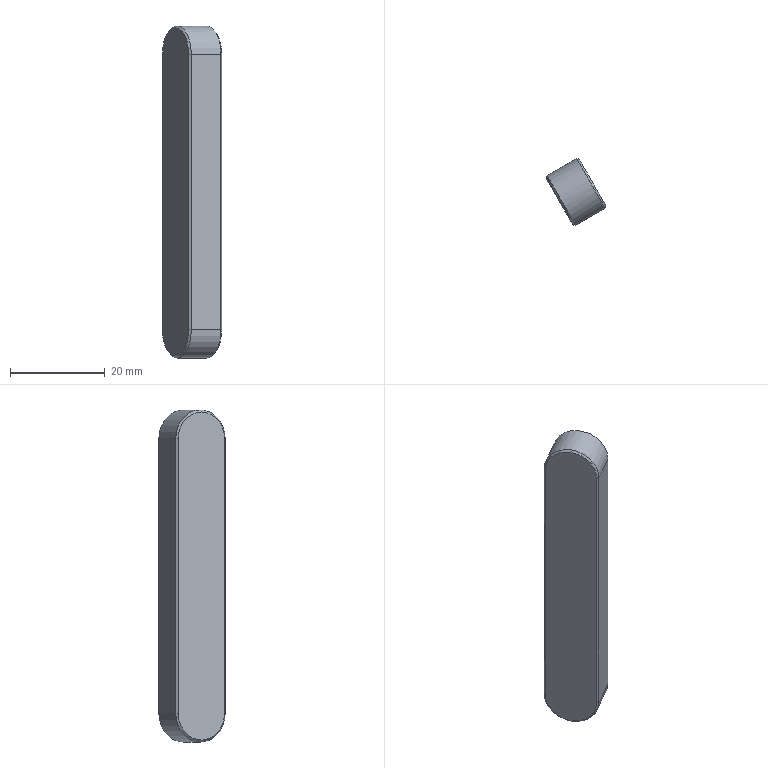Component | SolidWorks | Key12-8-70-1 | 1 solid | 17 faces | box 12.5 x 13.99 x 70 mm | volume 6448 mm3 | plane 8 | cone 6 | cylinder 3 | commonest cylinder face diameters 12 x3
build123d program:
from build123d import *

# Parameters (mm, degrees)
BOSS_EXTRUDE1_DEPTH = 8
CHAMFER1_SIZE2      = 0.4
CHAMFER1_SIZE       = 0.4


with BuildPart() as part:
    # Sketch1 → Boss-Extrude1 (new body)
    with BuildSketch(Plane(origin=(0, 0, 4), x_dir=(1, 0, 0), z_dir=(0, -1, 0))):
        with BuildLine():
            Line((-6, 54), (-6, -4))
            ThreePointArc((-6, -4), (0, -10), (6, -4))
            Line((6, -4), (6, 54))
            ThreePointArc((6, 54), (0, 60), (-6, 54))
        make_face()
    extrude(amount=-BOSS_EXTRUDE1_DEPTH)

    # Chamfer1
    chamfer1_edges = [part.edges().sort_by_distance(p)[0] for p in [
        (0, 8, -6),
        (6, 8, 29),
        (0, 8, 64),
        (6, 0, 29),
        (0, 0, -6),
        (-6, 0, 29),
        (0, 0, 64),
        (-6, 8, 29),
    ]]
    chamfer(chamfer1_edges, length=CHAMFER1_SIZE, length2=CHAMFER1_SIZE2)


solid = part.part

# Placed as in the assembly
solid = solid.moved(Location((-50.674, -11.79, -169.75), (-180, 0, -119.696)))
STEP:
#1=CARTESIAN_POINT('',(-1.721,-0.3082,-9.187));
#2=VERTEX_POINT('',#1);
#3=CARTESIAN_POINT('',(-1.831,-0.1166,-8.967));
#4=VERTEX_POINT('',#3);
#5=CARTESIAN_POINT('',(-1.721,-0.3082,-8.967));
#6=DIRECTION('',(0.8687,0.4954,0.));
#7=DIRECTION('',(0.,-0.,-1.));
#8=AXIS2_PLACEMENT_3D('',#5,#6,#7);
#9=CIRCLE('',#8,0.2205);
#10=EDGE_CURVE('',#2,#4,#9,.T.);
#11=ORIENTED_EDGE('',*,*,#10,.F.);
#12=CARTESIAN_POINT('',(-1.735,-0.316,-9.203));
#13=VERTEX_POINT('',#12);
#14=CARTESIAN_POINT('',(-1.735,-0.316,-9.203));
#15=DIRECTION('',(-0.6142,-0.3503,-0.7071));
#16=VECTOR('',#15,39.37);
#17=LINE('',#14,#16);
#18=EDGE_CURVE('',#2,#13,#17,.T.);
#19=ORIENTED_EDGE('',*,*,#18,.T.);
#20=CARTESIAN_POINT('',(-1.852,-0.1108,-8.967));
#21=VERTEX_POINT('',#20);
#22=CARTESIAN_POINT('',(-1.735,-0.316,-8.967));
#23=DIRECTION('',(-0.8687,-0.4954,-0.));
#24=DIRECTION('',(0.,0.,-1.));
#25=AXIS2_PLACEMENT_3D('',#22,#23,#24);
#26=CIRCLE('',#25,0.2362);
#27=EDGE_CURVE('',#21,#13,#26,.T.);
#28=ORIENTED_EDGE('',*,*,#27,.F.);
#29=CARTESIAN_POINT('',(-1.831,-0.1166,-8.967));
#30=DIRECTION('',(-0.9645,0.2639,-0.));
#31=VECTOR('',#30,39.37);
#32=LINE('',#29,#31);
#33=EDGE_CURVE('',#4,#21,#32,.T.);
#34=ORIENTED_EDGE('',*,*,#33,.F.);
#35=EDGE_LOOP('',(#11,#19,#28,#34));
#36=FACE_OUTER_BOUND('',#35,.T.);
#37=CARTESIAN_POINT('',(-1.735,-0.316,-8.967));
#38=DIRECTION('',(-0.8687,-0.4954,-0.));
#39=DIRECTION('',(0.,0.,-1.));
#40=AXIS2_PLACEMENT_3D('',#37,#38,#39);
#41=CONICAL_SURFACE('',#40,0.2362,0.7854);
#42=ADVANCED_FACE('',(#36),#41,.T.);
#43=CARTESIAN_POINT('',(-1.995,-0.4642,-6.463));
#44=VERTEX_POINT('',#43);
#45=CARTESIAN_POINT('',(-2.104,-0.2727,-6.683));
#46=VERTEX_POINT('',#45);
#47=CARTESIAN_POINT('',(-1.995,-0.4642,-6.683));
#48=DIRECTION('',(-0.8687,-0.4954,-0.));
#49=DIRECTION('',(0.,0.,-1.));
#50=AXIS2_PLACEMENT_3D('',#47,#48,#49);
#51=CIRCLE('',#50,0.2205);
#52=EDGE_CURVE('',#44,#46,#51,.T.);
#53=ORIENTED_EDGE('',*,*,#52,.F.);
#54=CARTESIAN_POINT('',(-1.981,-0.4564,-6.447));
#55=VERTEX_POINT('',#54);
#56=CARTESIAN_POINT('',(-1.995,-0.4642,-6.463));
#57=DIRECTION('',(0.6142,0.3503,0.7071));
#58=VECTOR('',#57,39.37);
#59=LINE('',#56,#58);
#60=EDGE_CURVE('',#44,#55,#59,.T.);
#61=ORIENTED_EDGE('',*,*,#60,.T.);
#62=CARTESIAN_POINT('',(-2.098,-0.2512,-6.683));
#63=VERTEX_POINT('',#62);
#64=CARTESIAN_POINT('',(-1.981,-0.4564,-6.683));
#65=DIRECTION('',(0.8687,0.4954,0.));
#66=DIRECTION('',(0.,0.,-1.));
#67=AXIS2_PLACEMENT_3D('',#64,#65,#66);
#68=CIRCLE('',#67,0.2362);
#69=EDGE_CURVE('',#63,#55,#68,.T.);
#70=ORIENTED_EDGE('',*,*,#69,.F.);
#71=CARTESIAN_POINT('',(-2.098,-0.2512,-6.683));
#72=DIRECTION('',(-0.2639,-0.9645,-0.));
#73=VECTOR('',#72,39.37);
#74=LINE('',#71,#73);
#75=EDGE_CURVE('',#63,#46,#74,.T.);
#76=ORIENTED_EDGE('',*,*,#75,.T.);
#77=EDGE_LOOP('',(#53,#61,#70,#76));
#78=FACE_OUTER_BOUND('',#77,.T.);
#79=CARTESIAN_POINT('',(-1.995,-0.4642,-6.683));
#80=DIRECTION('',(0.8687,0.4954,0.));
#81=DIRECTION('',(-0.,0.,1.));
#82=AXIS2_PLACEMENT_3D('',#79,#80,#81);
#83=CONICAL_SURFACE('',#82,0.2205,0.7854);
#84=ADVANCED_FACE('',(#78),#83,.T.);
#85=ORIENTED_EDGE('',*,*,#27,.T.);
#86=CARTESIAN_POINT('',(-1.981,-0.4564,-9.203));
#87=VERTEX_POINT('',#86);
#88=CARTESIAN_POINT('',(-1.721,-0.3082,-9.203));
#89=DIRECTION('',(-0.8687,-0.4954,-0.));
#90=VECTOR('',#89,39.37);
#91=LINE('',#88,#90);
#92=EDGE_CURVE('',#13,#87,#91,.T.);
#93=ORIENTED_EDGE('',*,*,#92,.T.);
#94=CARTESIAN_POINT('',(-2.098,-0.2512,-8.967));
#95=VERTEX_POINT('',#94);
#96=CARTESIAN_POINT('',(-1.981,-0.4564,-8.967));
#97=DIRECTION('',(0.8687,0.4954,0.));
#98=DIRECTION('',(0.,0.,-1.));
#99=AXIS2_PLACEMENT_3D('',#96,#97,#98);
#100=CIRCLE('',#99,0.2362);
#101=EDGE_CURVE('',#87,#95,#100,.T.);
#102=ORIENTED_EDGE('',*,*,#101,.T.);
#103=CARTESIAN_POINT('',(-1.838,-0.103,-8.967));
#104=DIRECTION('',(-0.8687,-0.4954,-0.));
#105=VECTOR('',#104,39.37);
#106=LINE('',#103,#105);
#107=EDGE_CURVE('',#21,#95,#106,.T.);
#108=ORIENTED_EDGE('',*,*,#107,.F.);
#109=EDGE_LOOP('',(#85,#93,#102,#108));
#110=FACE_OUTER_BOUND('',#109,.T.);
#111=CARTESIAN_POINT('',(-1.721,-0.3082,-8.967));
#112=DIRECTION('',(-0.8687,-0.4954,-0.));
#113=DIRECTION('',(0.,0.,-1.));
#114=AXIS2_PLACEMENT_3D('',#111,#112,#113);
#115=CYLINDRICAL_SURFACE('',#114,0.2362);
#116=ADVANCED_FACE('',(#110),#115,.T.);
#117=CARTESIAN_POINT('',(-1.852,-0.1108,-6.683));
#118=VERTEX_POINT('',#117);
#119=CARTESIAN_POINT('',(-1.838,-0.103,-6.683));
#120=DIRECTION('',(-0.8687,-0.4954,-0.));
#121=VECTOR('',#120,39.37);
#122=LINE('',#119,#121);
#123=EDGE_CURVE('',#118,#63,#122,.T.);
#124=ORIENTED_EDGE('',*,*,#123,.T.);
#125=ORIENTED_EDGE('',*,*,#69,.T.);
#126=CARTESIAN_POINT('',(-1.864,-0.6616,-6.683));
#127=VERTEX_POINT('',#126);
#128=CARTESIAN_POINT('',(-1.981,-0.4564,-6.683));
#129=DIRECTION('',(0.8687,0.4954,0.));
#130=DIRECTION('',(0.,-0.,-1.));
#131=AXIS2_PLACEMENT_3D('',#128,#129,#130);
#132=CIRCLE('',#131,0.2362);
#133=EDGE_CURVE('',#55,#127,#132,.T.);
#134=ORIENTED_EDGE('',*,*,#133,.T.);
#135=CARTESIAN_POINT('',(-1.618,-0.5212,-6.683));
#136=VERTEX_POINT('',#135);
#137=CARTESIAN_POINT('',(-1.604,-0.5134,-6.683));
#138=DIRECTION('',(-0.8687,-0.4954,-0.));
#139=VECTOR('',#138,39.37);
#140=LINE('',#137,#139);
#141=EDGE_CURVE('',#136,#127,#140,.T.);
#142=ORIENTED_EDGE('',*,*,#141,.F.);
#143=CARTESIAN_POINT('',(-1.735,-0.316,-6.683));
#144=DIRECTION('',(-0.8687,-0.4954,-0.));
#145=DIRECTION('',(0.,0.,-1.));
#146=AXIS2_PLACEMENT_3D('',#143,#144,#145);
#147=CIRCLE('',#146,0.2362);
#148=EDGE_CURVE('',#136,#118,#147,.T.);
#149=ORIENTED_EDGE('',*,*,#148,.T.);
#150=EDGE_LOOP('',(#124,#125,#134,#142,#149));
#151=FACE_OUTER_BOUND('',#150,.T.);
#152=CARTESIAN_POINT('',(-1.721,-0.3082,-6.683));
#153=DIRECTION('',(-0.8687,-0.4954,-0.));
#154=DIRECTION('',(0.,0.,-1.));
#155=AXIS2_PLACEMENT_3D('',#152,#153,#154);
#156=CYLINDRICAL_SURFACE('',#155,0.2362);
#157=ADVANCED_FACE('',(#151),#156,.T.);
#158=ORIENTED_EDGE('',*,*,#141,.T.);
#159=CARTESIAN_POINT('',(-1.864,-0.6616,-8.967));
#160=VERTEX_POINT('',#159);
#161=CARTESIAN_POINT('',(-1.864,-0.6616,-8.967));
#162=DIRECTION('',(0.,0.,-1.));
#163=VECTOR('',#162,39.37);
#164=LINE('',#161,#163);
#165=EDGE_CURVE('',#127,#160,#164,.T.);
#166=ORIENTED_EDGE('',*,*,#165,.T.);
#167=CARTESIAN_POINT('',(-1.618,-0.5212,-8.967));
#168=VERTEX_POINT('',#167);
#169=CARTESIAN_POINT('',(-1.604,-0.5134,-8.967));
#170=DIRECTION('',(-0.8687,-0.4954,-0.));
#171=VECTOR('',#170,39.37);
#172=LINE('',#169,#171);
#173=EDGE_CURVE('',#168,#160,#172,.T.);
#174=ORIENTED_EDGE('',*,*,#173,.F.);
#175=CARTESIAN_POINT('',(-1.618,-0.5212,-6.683));
#176=DIRECTION('',(-0.,-0.,1.));
#177=VECTOR('',#176,39.37);
#178=LINE('',#175,#177);
#179=EDGE_CURVE('',#168,#136,#178,.T.);
#180=ORIENTED_EDGE('',*,*,#179,.T.);
#181=EDGE_LOOP('',(#158,#166,#174,#180));
#182=FACE_OUTER_BOUND('',#181,.T.);
#183=CARTESIAN_POINT('',(-1.604,-0.5134,-8.967));
#184=DIRECTION('',(0.4954,-0.8687,0.));
#185=DIRECTION('',(0.,0.,-1.));
#186=AXIS2_PLACEMENT_3D('',#183,#184,#185);
#187=PLANE('',#186);
#188=ADVANCED_FACE('',(#182),#187,.T.);
#189=ORIENTED_EDGE('',*,*,#92,.F.);
#190=CARTESIAN_POINT('',(-1.735,-0.316,-8.967));
#191=DIRECTION('',(-0.8687,-0.4954,-0.));
#192=DIRECTION('',(0.,0.,-1.));
#193=AXIS2_PLACEMENT_3D('',#190,#191,#192);
#194=CIRCLE('',#193,0.2362);
#195=EDGE_CURVE('',#13,#168,#194,.T.);
#196=ORIENTED_EDGE('',*,*,#195,.T.);
#197=ORIENTED_EDGE('',*,*,#173,.T.);
#198=CARTESIAN_POINT('',(-1.981,-0.4564,-8.967));
#199=DIRECTION('',(0.8687,0.4954,0.));
#200=DIRECTION('',(0.,0.,-1.));
#201=AXIS2_PLACEMENT_3D('',#198,#199,#200);
#202=CIRCLE('',#201,0.2362);
#203=EDGE_CURVE('',#160,#87,#202,.T.);
#204=ORIENTED_EDGE('',*,*,#203,.T.);
#205=EDGE_LOOP('',(#189,#196,#197,#204));
#206=FACE_OUTER_BOUND('',#205,.T.);
#207=CARTESIAN_POINT('',(-1.721,-0.3082,-8.967));
#208=DIRECTION('',(-0.8687,-0.4954,-0.));
#209=DIRECTION('',(0.,0.,-1.));
#210=AXIS2_PLACEMENT_3D('',#207,#208,#209);
#211=CYLINDRICAL_SURFACE('',#210,0.2362);
#212=ADVANCED_FACE('',(#206),#211,.T.);
#213=ORIENTED_EDGE('',*,*,#107,.T.);
#214=CARTESIAN_POINT('',(-2.098,-0.2512,-6.683));
#215=DIRECTION('',(-0.,-0.,1.));
#216=VECTOR('',#215,39.37);
#217=LINE('',#214,#216);
#218=EDGE_CURVE('',#95,#63,#217,.T.);
#219=ORIENTED_EDGE('',*,*,#218,.T.);
#220=ORIENTED_EDGE('',*,*,#123,.F.);
#221=CARTESIAN_POINT('',(-1.852,-0.1108,-8.967));
#222=DIRECTION('',(0.,0.,-1.));
#223=VECTOR('',#222,39.37);
#224=LINE('',#221,#223);
#225=EDGE_CURVE('',#118,#21,#224,.T.);
#226=ORIENTED_EDGE('',*,*,#225,.T.);
#227=EDGE_LOOP('',(#213,#219,#220,#226));
#228=FACE_OUTER_BOUND('',#227,.T.);
#229=CARTESIAN_POINT('',(-1.838,-0.103,-6.683));
#230=DIRECTION('',(-0.4954,0.8687,-0.));
#231=DIRECTION('',(-0.,-0.,1.));
#232=AXIS2_PLACEMENT_3D('',#229,#230,#231);
#233=PLANE('',#232);
#234=ADVANCED_FACE('',(#228),#233,.T.);
#235=CARTESIAN_POINT('',(-1.612,-0.4997,-8.967));
#236=VERTEX_POINT('',#235);
#237=CARTESIAN_POINT('',(-1.721,-0.3082,-8.967));
#238=DIRECTION('',(0.8687,0.4954,0.));
#239=DIRECTION('',(0.,0.,-1.));
#240=AXIS2_PLACEMENT_3D('',#237,#238,#239);
#241=CIRCLE('',#240,0.2205);
#242=EDGE_CURVE('',#236,#2,#241,.T.);
#243=ORIENTED_EDGE('',*,*,#242,.T.);
#244=ORIENTED_EDGE('',*,*,#10,.T.);
#245=CARTESIAN_POINT('',(-1.831,-0.1166,-6.683));
#246=VERTEX_POINT('',#245);
#247=CARTESIAN_POINT('',(-1.831,-0.1166,-6.683));
#248=DIRECTION('',(-0.,-0.,1.));
#249=VECTOR('',#248,39.37);
#250=LINE('',#247,#249);
#251=EDGE_CURVE('',#4,#246,#250,.T.);
#252=ORIENTED_EDGE('',*,*,#251,.T.);
#253=CARTESIAN_POINT('',(-1.612,-0.4997,-6.683));
#254=VERTEX_POINT('',#253);
#255=CARTESIAN_POINT('',(-1.721,-0.3082,-6.683));
#256=DIRECTION('',(0.8687,0.4954,0.));
#257=DIRECTION('',(0.,0.,-1.));
#258=AXIS2_PLACEMENT_3D('',#255,#256,#257);
#259=CIRCLE('',#258,0.2205);
#260=EDGE_CURVE('',#246,#254,#259,.T.);
#261=ORIENTED_EDGE('',*,*,#260,.T.);
#262=CARTESIAN_POINT('',(-1.612,-0.4997,-8.967));
#263=DIRECTION('',(0.,0.,-1.));
#264=VECTOR('',#263,39.37);
#265=LINE('',#262,#264);
#266=EDGE_CURVE('',#254,#236,#265,.T.);
#267=ORIENTED_EDGE('',*,*,#266,.T.);
#268=EDGE_LOOP('',(#243,#244,#252,#261,#267));
#269=FACE_OUTER_BOUND('',#268,.T.);
#270=CARTESIAN_POINT('',(-1.721,-0.3082,-6.683));
#271=DIRECTION('',(-0.8687,-0.4954,-0.));
#272=DIRECTION('',(0.,0.,-1.));
#273=AXIS2_PLACEMENT_3D('',#270,#271,#272);
#274=PLANE('',#273);
#275=ADVANCED_FACE('',(#269),#274,.F.);
#276=CARTESIAN_POINT('',(-2.104,-0.2727,-8.967));
#277=VERTEX_POINT('',#276);
#278=CARTESIAN_POINT('',(-1.886,-0.6557,-8.967));
#279=VERTEX_POINT('',#278);
#280=CARTESIAN_POINT('',(-1.995,-0.4642,-8.967));
#281=DIRECTION('',(-0.8687,-0.4954,-0.));
#282=DIRECTION('',(0.,0.,-1.));
#283=AXIS2_PLACEMENT_3D('',#280,#281,#282);
#284=CIRCLE('',#283,0.2205);
#285=EDGE_CURVE('',#277,#279,#284,.T.);
#286=ORIENTED_EDGE('',*,*,#285,.T.);
#287=CARTESIAN_POINT('',(-1.886,-0.6557,-6.683));
#288=VERTEX_POINT('',#287);
#289=CARTESIAN_POINT('',(-1.886,-0.6557,-6.683));
#290=DIRECTION('',(-0.,-0.,1.));
#291=VECTOR('',#290,39.37);
#292=LINE('',#289,#291);
#293=EDGE_CURVE('',#279,#288,#292,.T.);
#294=ORIENTED_EDGE('',*,*,#293,.T.);
#295=CARTESIAN_POINT('',(-1.995,-0.4642,-6.683));
#296=DIRECTION('',(-0.8687,-0.4954,-0.));
#297=DIRECTION('',(0.,0.,-1.));
#298=AXIS2_PLACEMENT_3D('',#295,#296,#297);
#299=CIRCLE('',#298,0.2205);
#300=EDGE_CURVE('',#288,#44,#299,.T.);
#301=ORIENTED_EDGE('',*,*,#300,.T.);
#302=ORIENTED_EDGE('',*,*,#52,.T.);
#303=CARTESIAN_POINT('',(-2.104,-0.2727,-6.683));
#304=DIRECTION('',(0.,0.,-1.));
#305=VECTOR('',#304,39.37);
#306=LINE('',#303,#305);
#307=EDGE_CURVE('',#46,#277,#306,.T.);
#308=ORIENTED_EDGE('',*,*,#307,.T.);
#309=EDGE_LOOP('',(#286,#294,#301,#302,#308));
#310=FACE_OUTER_BOUND('',#309,.T.);
#311=CARTESIAN_POINT('',(-1.995,-0.4642,-6.683));
#312=DIRECTION('',(-0.8687,-0.4954,-0.));
#313=DIRECTION('',(0.,0.,-1.));
#314=AXIS2_PLACEMENT_3D('',#311,#312,#313);
#315=PLANE('',#314);
#316=ADVANCED_FACE('',(#310),#315,.T.);
#317=ORIENTED_EDGE('',*,*,#75,.F.);
#318=ORIENTED_EDGE('',*,*,#218,.F.);
#319=CARTESIAN_POINT('',(-2.104,-0.2727,-8.967));
#320=DIRECTION('',(0.2639,0.9645,0.));
#321=VECTOR('',#320,39.37);
#322=LINE('',#319,#321);
#323=EDGE_CURVE('',#277,#95,#322,.T.);
#324=ORIENTED_EDGE('',*,*,#323,.F.);
#325=ORIENTED_EDGE('',*,*,#307,.F.);
#326=EDGE_LOOP('',(#317,#318,#324,#325));
#327=FACE_OUTER_BOUND('',#326,.T.);
#328=CARTESIAN_POINT('',(-2.104,-0.2727,-6.683));
#329=DIRECTION('',(0.9645,-0.2639,0.));
#330=DIRECTION('',(0.,0.,-1.));
#331=AXIS2_PLACEMENT_3D('',#328,#329,#330);
#332=PLANE('',#331);
#333=ADVANCED_FACE('',(#327),#332,.F.);
#334=ORIENTED_EDGE('',*,*,#323,.T.);
#335=ORIENTED_EDGE('',*,*,#101,.F.);
#336=ORIENTED_EDGE('',*,*,#203,.F.);
#337=CARTESIAN_POINT('',(-1.886,-0.6557,-8.967));
#338=DIRECTION('',(0.9645,-0.2639,0.));
#339=VECTOR('',#338,39.37);
#340=LINE('',#337,#339);
#341=EDGE_CURVE('',#279,#160,#340,.T.);
#342=ORIENTED_EDGE('',*,*,#341,.F.);
#343=ORIENTED_EDGE('',*,*,#285,.F.);
#344=EDGE_LOOP('',(#334,#335,#336,#342,#343));
#345=FACE_OUTER_BOUND('',#344,.T.);
#346=CARTESIAN_POINT('',(-1.995,-0.4642,-8.967));
#347=DIRECTION('',(0.8687,0.4954,0.));
#348=DIRECTION('',(-0.,0.,1.));
#349=AXIS2_PLACEMENT_3D('',#346,#347,#348);
#350=CONICAL_SURFACE('',#349,0.2205,0.7854);
#351=ADVANCED_FACE('',(#345),#350,.T.);
#352=ORIENTED_EDGE('',*,*,#60,.F.);
#353=ORIENTED_EDGE('',*,*,#300,.F.);
#354=CARTESIAN_POINT('',(-1.864,-0.6616,-6.683));
#355=DIRECTION('',(-0.9645,0.2639,-0.));
#356=VECTOR('',#355,39.37);
#357=LINE('',#354,#356);
#358=EDGE_CURVE('',#127,#288,#357,.T.);
#359=ORIENTED_EDGE('',*,*,#358,.F.);
#360=ORIENTED_EDGE('',*,*,#133,.F.);
#361=EDGE_LOOP('',(#352,#353,#359,#360));
#362=FACE_OUTER_BOUND('',#361,.T.);
#363=CARTESIAN_POINT('',(-1.995,-0.4642,-6.683));
#364=DIRECTION('',(0.8687,0.4954,0.));
#365=DIRECTION('',(-0.,0.,1.));
#366=AXIS2_PLACEMENT_3D('',#363,#364,#365);
#367=CONICAL_SURFACE('',#366,0.2205,0.7854);
#368=ADVANCED_FACE('',(#362),#367,.T.);
#369=ORIENTED_EDGE('',*,*,#341,.T.);
#370=ORIENTED_EDGE('',*,*,#165,.F.);
#371=ORIENTED_EDGE('',*,*,#358,.T.);
#372=ORIENTED_EDGE('',*,*,#293,.F.);
#373=EDGE_LOOP('',(#369,#370,#371,#372));
#374=FACE_OUTER_BOUND('',#373,.T.);
#375=CARTESIAN_POINT('',(-1.886,-0.6557,-6.683));
#376=DIRECTION('',(0.2639,0.9645,0.));
#377=DIRECTION('',(-0.,-0.,1.));
#378=AXIS2_PLACEMENT_3D('',#375,#376,#377);
#379=PLANE('',#378);
#380=ADVANCED_FACE('',(#374),#379,.F.);
#381=CARTESIAN_POINT('',(-1.612,-0.4997,-8.967));
#382=DIRECTION('',(-0.2639,-0.9645,-0.));
#383=VECTOR('',#382,39.37);
#384=LINE('',#381,#383);
#385=EDGE_CURVE('',#236,#168,#384,.T.);
#386=ORIENTED_EDGE('',*,*,#385,.F.);
#387=ORIENTED_EDGE('',*,*,#266,.F.);
#388=CARTESIAN_POINT('',(-1.618,-0.5212,-6.683));
#389=DIRECTION('',(0.2639,0.9645,0.));
#390=VECTOR('',#389,39.37);
#391=LINE('',#388,#390);
#392=EDGE_CURVE('',#136,#254,#391,.T.);
#393=ORIENTED_EDGE('',*,*,#392,.F.);
#394=ORIENTED_EDGE('',*,*,#179,.F.);
#395=EDGE_LOOP('',(#386,#387,#393,#394));
#396=FACE_OUTER_BOUND('',#395,.T.);
#397=CARTESIAN_POINT('',(-1.618,-0.5212,-8.967));
#398=DIRECTION('',(0.9645,-0.2639,0.));
#399=DIRECTION('',(0.,0.,-1.));
#400=AXIS2_PLACEMENT_3D('',#397,#398,#399);
#401=PLANE('',#400);
#402=ADVANCED_FACE('',(#396),#401,.T.);
#403=ORIENTED_EDGE('',*,*,#392,.T.);
#404=ORIENTED_EDGE('',*,*,#260,.F.);
#405=CARTESIAN_POINT('',(-1.852,-0.1108,-6.683));
#406=DIRECTION('',(0.9645,-0.2639,0.));
#407=VECTOR('',#406,39.37);
#408=LINE('',#405,#407);
#409=EDGE_CURVE('',#118,#246,#408,.T.);
#410=ORIENTED_EDGE('',*,*,#409,.F.);
#411=ORIENTED_EDGE('',*,*,#148,.F.);
#412=EDGE_LOOP('',(#403,#404,#410,#411));
#413=FACE_OUTER_BOUND('',#412,.T.);
#414=CARTESIAN_POINT('',(-1.735,-0.316,-6.683));
#415=DIRECTION('',(-0.8687,-0.4954,-0.));
#416=DIRECTION('',(0.,0.,-1.));
#417=AXIS2_PLACEMENT_3D('',#414,#415,#416);
#418=CONICAL_SURFACE('',#417,0.2362,0.7854);
#419=ADVANCED_FACE('',(#413),#418,.T.);
#420=ORIENTED_EDGE('',*,*,#18,.F.);
#421=ORIENTED_EDGE('',*,*,#242,.F.);
#422=ORIENTED_EDGE('',*,*,#385,.T.);
#423=ORIENTED_EDGE('',*,*,#195,.F.);
#424=EDGE_LOOP('',(#420,#421,#422,#423));
#425=FACE_OUTER_BOUND('',#424,.T.);
#426=CARTESIAN_POINT('',(-1.735,-0.316,-8.967));
#427=DIRECTION('',(-0.8687,-0.4954,-0.));
#428=DIRECTION('',(0.,0.,-1.));
#429=AXIS2_PLACEMENT_3D('',#426,#427,#428);
#430=CONICAL_SURFACE('',#429,0.2362,0.7854);
#431=ADVANCED_FACE('',(#425),#430,.T.);
#432=ORIENTED_EDGE('',*,*,#409,.T.);
#433=ORIENTED_EDGE('',*,*,#251,.F.);
#434=ORIENTED_EDGE('',*,*,#33,.T.);
#435=ORIENTED_EDGE('',*,*,#225,.F.);
#436=EDGE_LOOP('',(#432,#433,#434,#435));
#437=FACE_OUTER_BOUND('',#436,.T.);
#438=CARTESIAN_POINT('',(-1.852,-0.1108,-6.683));
#439=DIRECTION('',(0.2639,0.9645,0.));
#440=DIRECTION('',(-0.,-0.,1.));
#441=AXIS2_PLACEMENT_3D('',#438,#439,#440);
#442=PLANE('',#441);
#443=ADVANCED_FACE('',(#437),#442,.T.);
#444=CLOSED_SHELL('',(#42,#84,#116,#157,#188,#212,#234,#275,#316,#333,#351,#368,#380,#402,#419,#431,#443));
#445=MANIFOLD_SOLID_BREP('',#444);
#446=CARTESIAN_POINT('',(0.,0.,0.));
#447=DIRECTION('',(0.,0.,1.));
#448=DIRECTION('',(1.,0.,0.));
#449=AXIS2_PLACEMENT_3D('',#446,#447,#448);
#450=(LENGTH_UNIT()NAMED_UNIT(*)SI_UNIT($,.METRE.));
#451=LENGTH_MEASURE_WITH_UNIT(LENGTH_MEASURE(0.0254),#450);
#452=DIMENSIONAL_EXPONENTS(1.,0.,0.,0.,0.,0.,0.);
#453=(CONVERSION_BASED_UNIT('',#451)LENGTH_UNIT()NAMED_UNIT(#452));
#454=UNCERTAINTY_MEASURE_WITH_UNIT(LENGTH_MEASURE(0.00001),#453,'','');
#455=(NAMED_UNIT(*)PLANE_ANGLE_UNIT()SI_UNIT($,.RADIAN.));
#456=(NAMED_UNIT(*)SI_UNIT($,.STERADIAN.)SOLID_ANGLE_UNIT());
#457=(GEOMETRIC_REPRESENTATION_CONTEXT(3)GLOBAL_UNCERTAINTY_ASSIGNED_CONTEXT((#454))GLOBAL_UNIT_ASSIGNED_CONTEXT((#453,#455,#456))REPRESENTATION_CONTEXT('',''));
#458=ADVANCED_BREP_SHAPE_REPRESENTATION('',(#445,#449),#457);
#459=COLOUR_RGB('',0.7922,0.8196,0.9333);
#460=FILL_AREA_STYLE_COLOUR('',#459);
#461=FILL_AREA_STYLE('',(#460));
#462=SURFACE_STYLE_FILL_AREA(#461);
#463=SURFACE_SIDE_STYLE('',(#462));
#464=SURFACE_STYLE_USAGE(.BOTH.,#463);
#465=PRESENTATION_STYLE_ASSIGNMENT((#464));
#466=STYLED_ITEM('',(#465),#445);
#467=PRESENTATION_LAYER_ASSIGNMENT('','',(#466));
#468=(LENGTH_UNIT()NAMED_UNIT(*)SI_UNIT($,.METRE.));
#469=LENGTH_MEASURE_WITH_UNIT(LENGTH_MEASURE(0.0254),#468);
#470=DIMENSIONAL_EXPONENTS(1.,0.,0.,0.,0.,0.,0.);
#471=(CONVERSION_BASED_UNIT('',#469)LENGTH_UNIT()NAMED_UNIT(#470));
#472=UNCERTAINTY_MEASURE_WITH_UNIT(LENGTH_MEASURE(0.00001),#471,'','');
#473=(NAMED_UNIT(*)PLANE_ANGLE_UNIT()SI_UNIT($,.RADIAN.));
#474=(NAMED_UNIT(*)SI_UNIT($,.STERADIAN.)SOLID_ANGLE_UNIT());
#475=(GEOMETRIC_REPRESENTATION_CONTEXT(3)GLOBAL_UNCERTAINTY_ASSIGNED_CONTEXT((#472))GLOBAL_UNIT_ASSIGNED_CONTEXT((#471,#473,#474))REPRESENTATION_CONTEXT('',''));
#476=MECHANICAL_DESIGN_GEOMETRIC_PRESENTATION_REPRESENTATION('',(#466),#475);